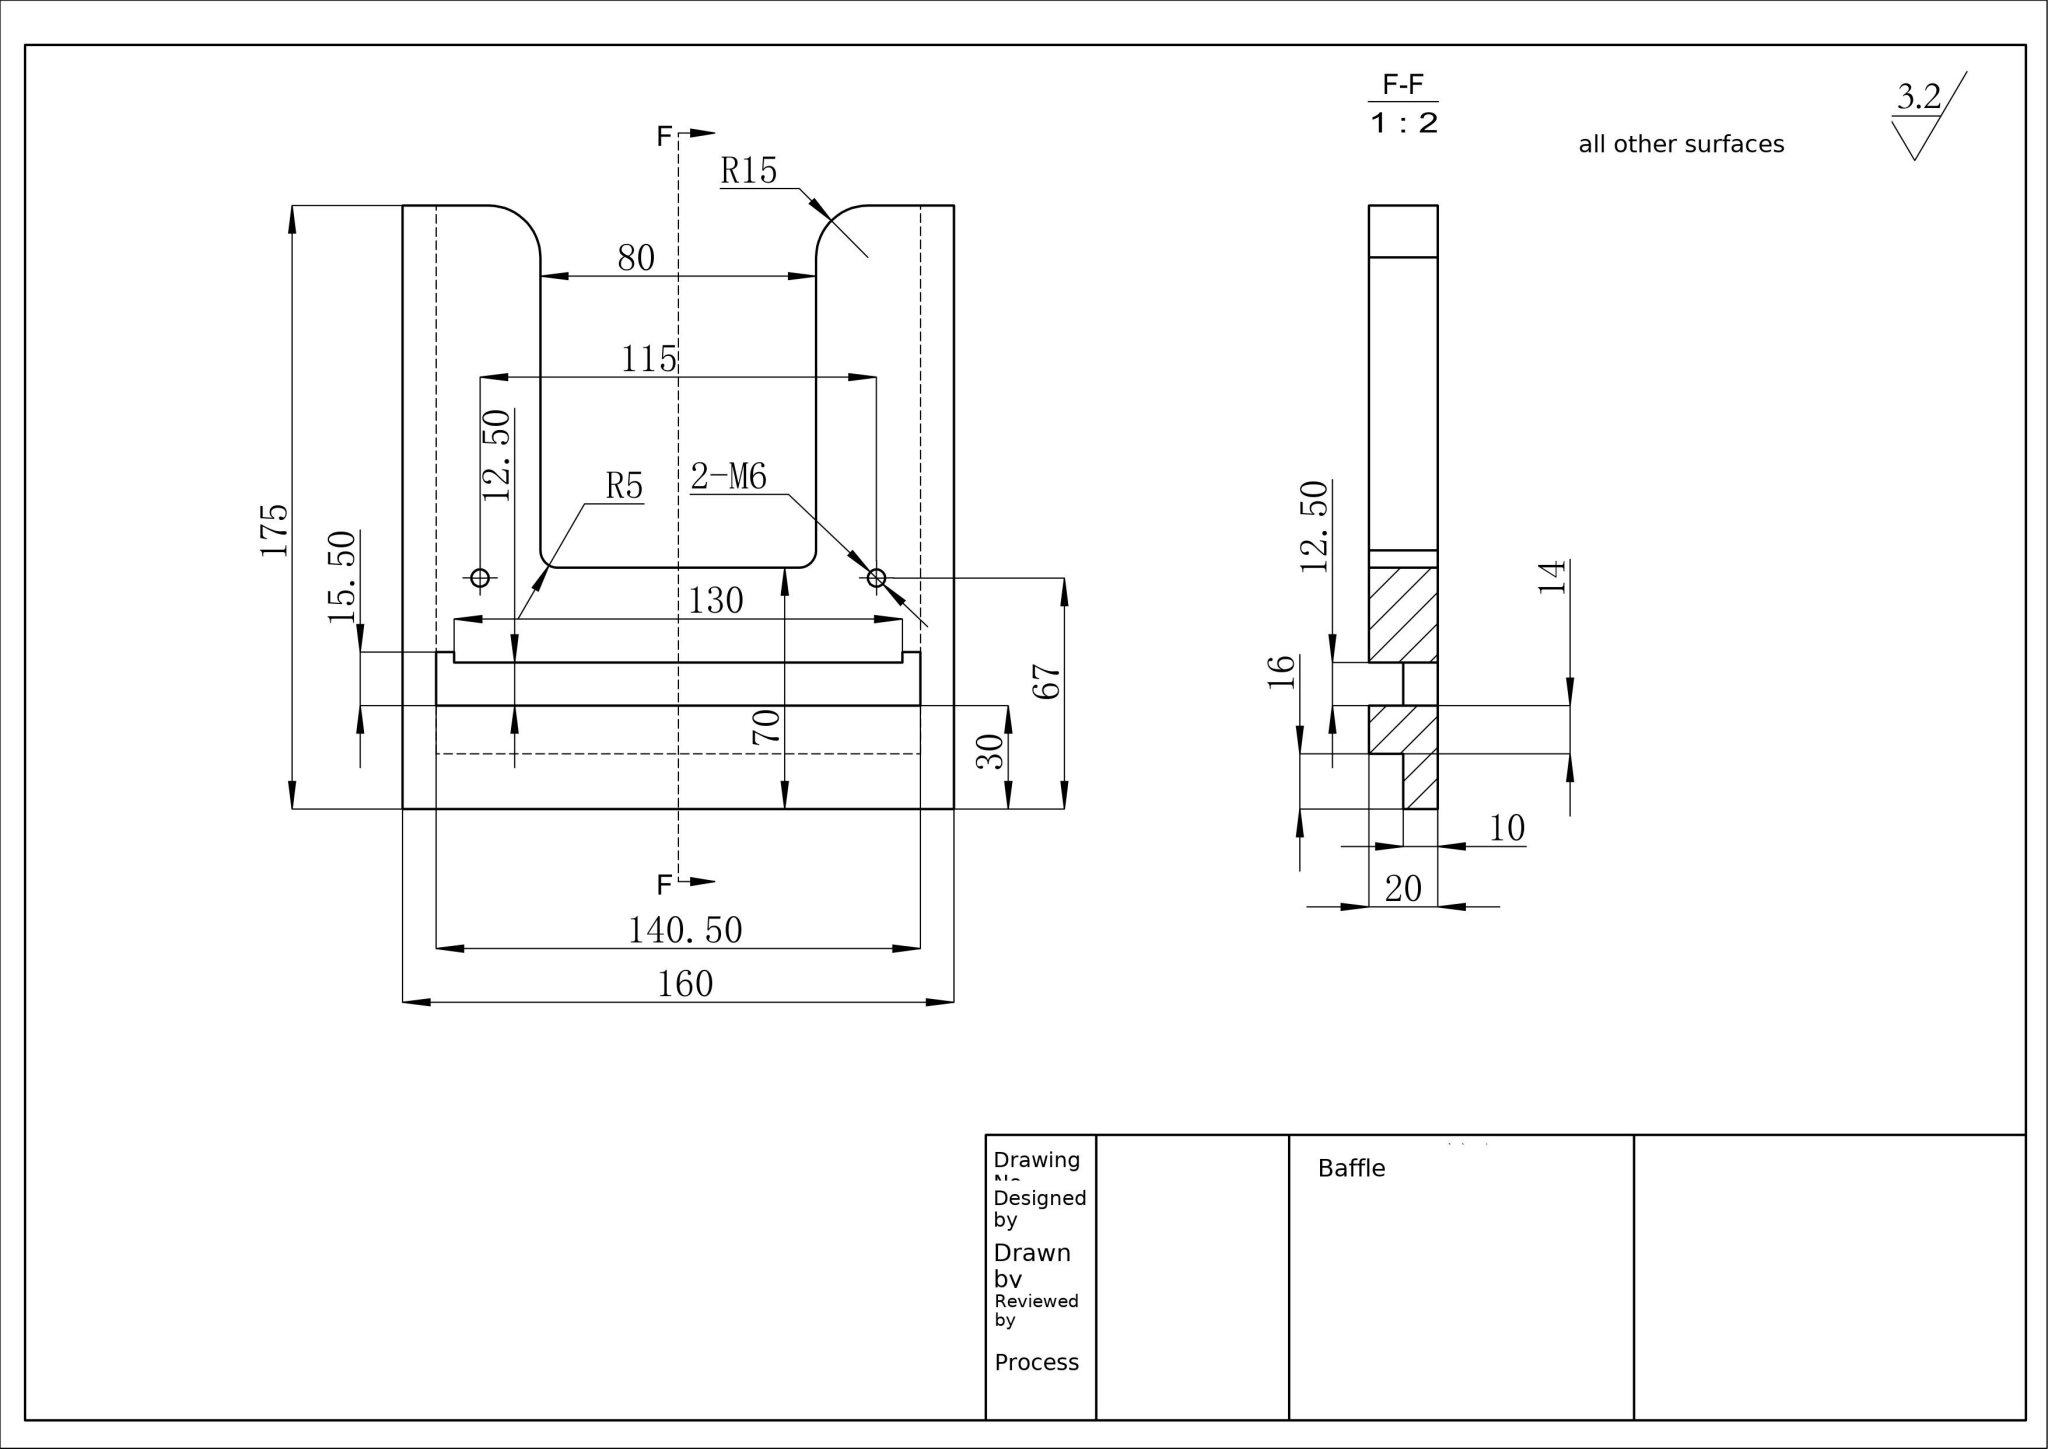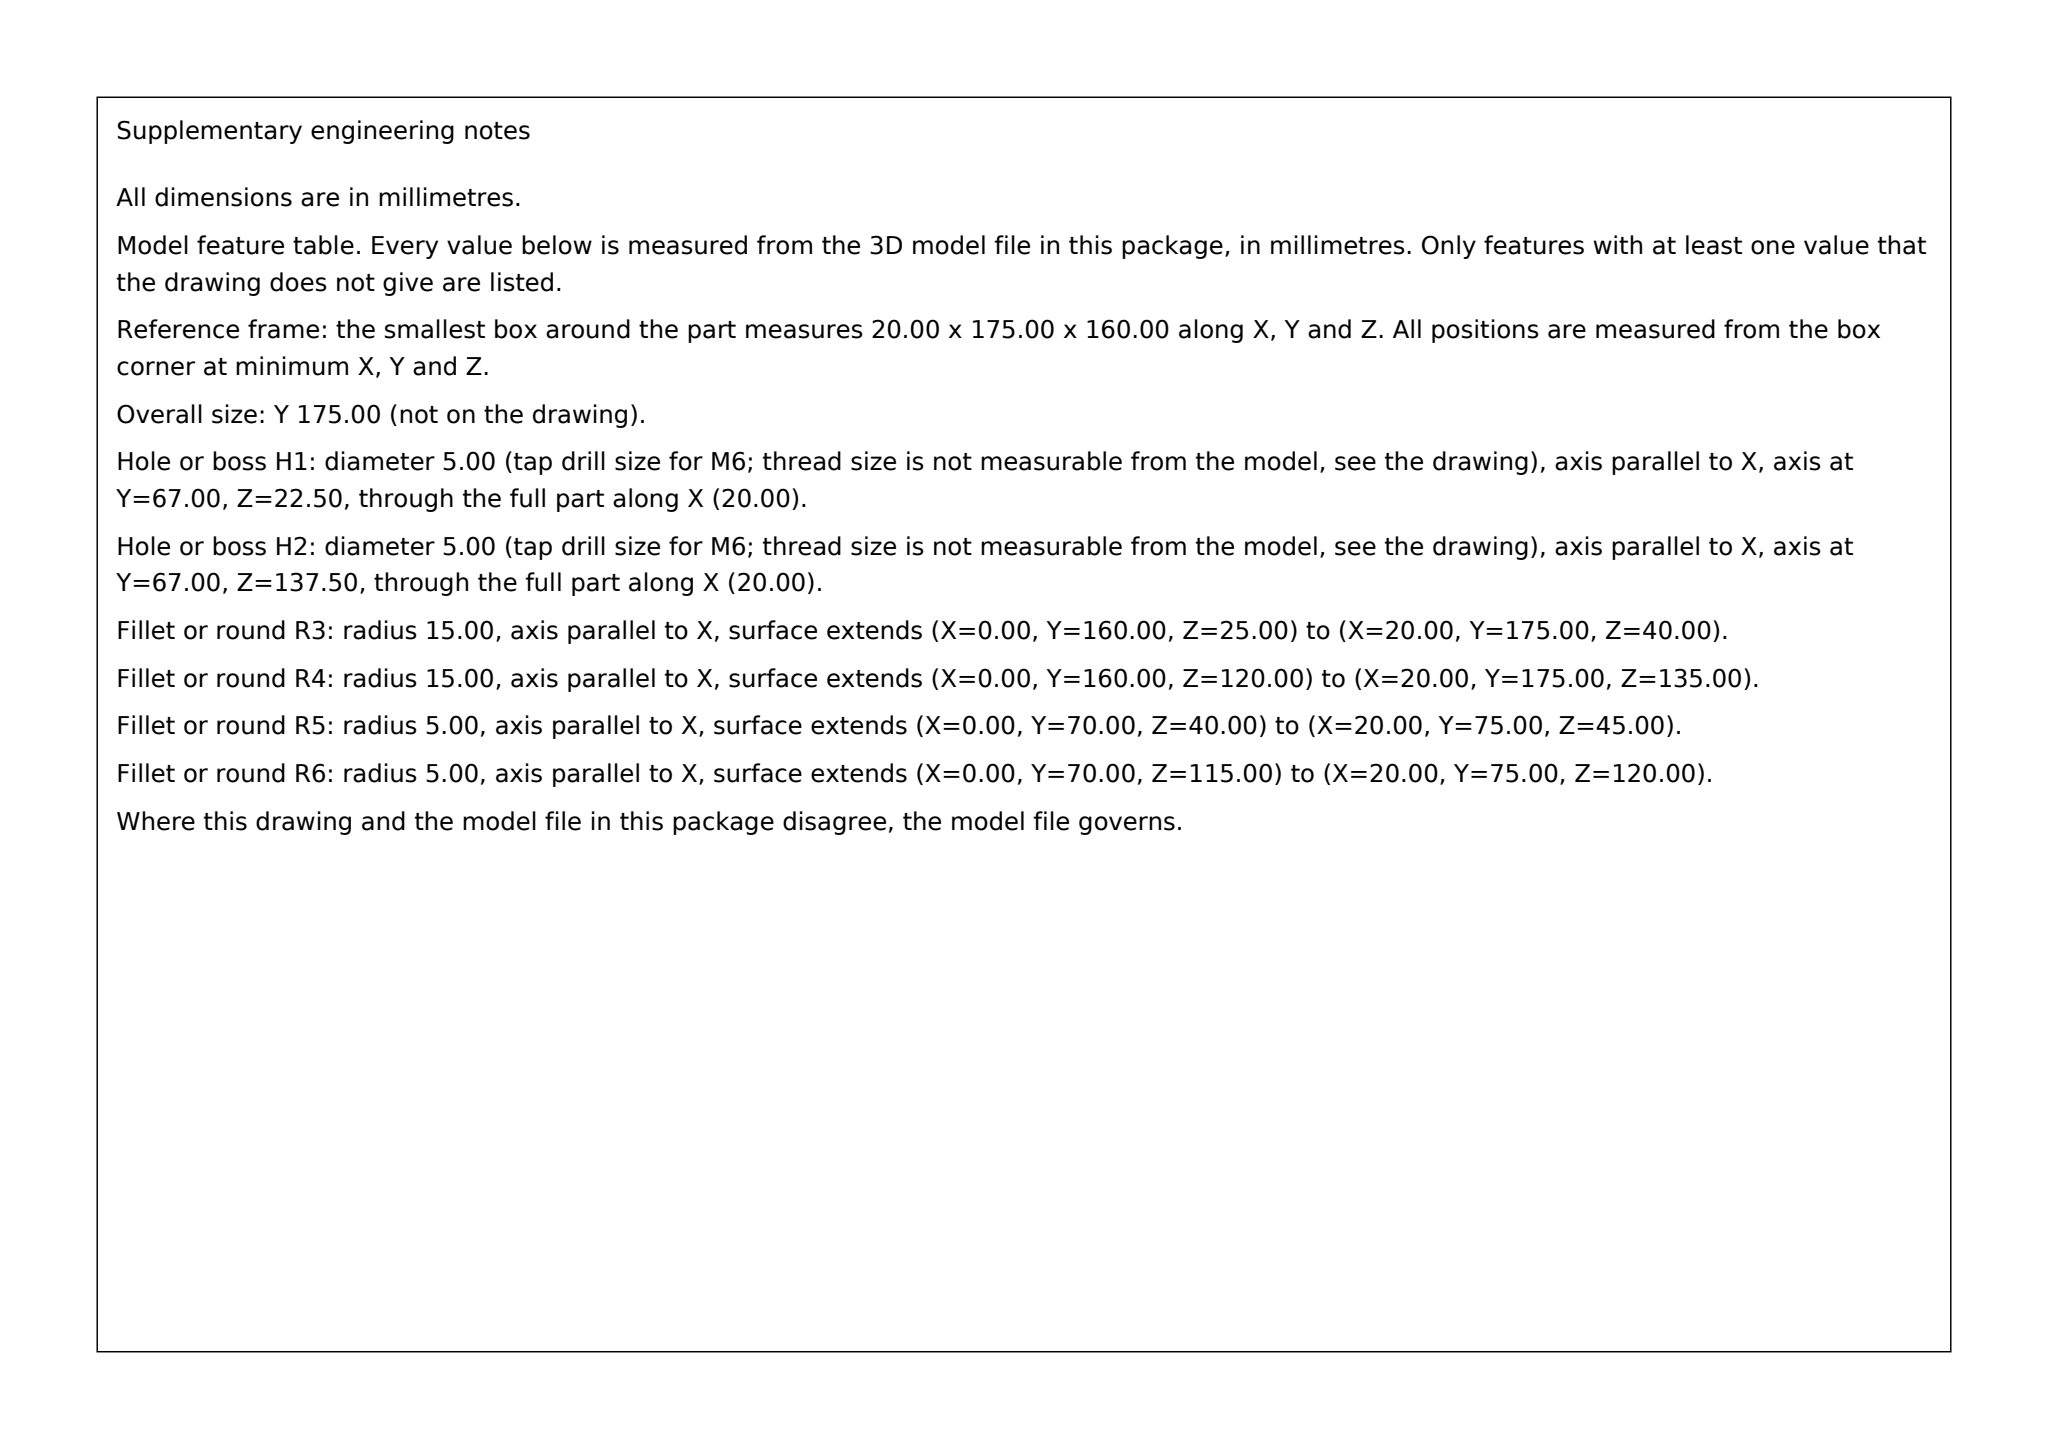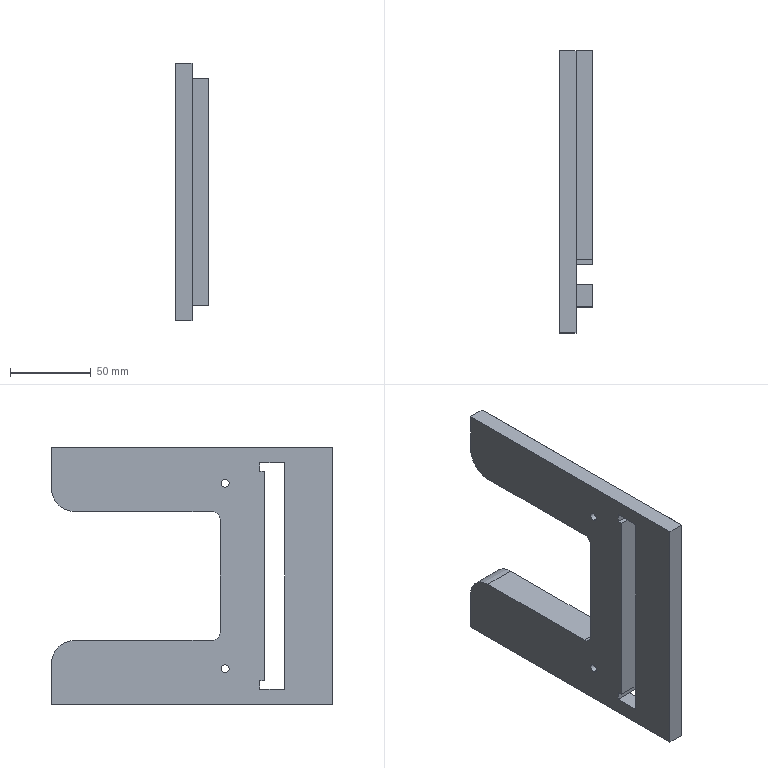Part | SolidWorks | mm | 1 solid | 33 faces | box 20 x 175 x 160 mm | volume 297138 mm3 | plane 25 | cylinder 8 | commonest cylinder face diameters 5 x4 30 x2 10 x2